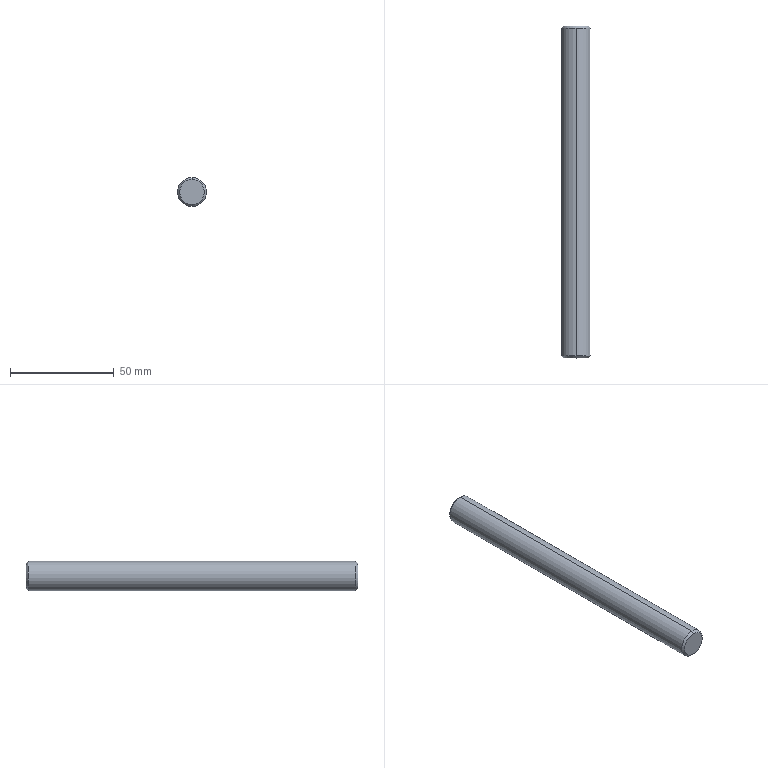Component | SolidWorks | AdjustingScrew9.26-3 | 1 solid | 8 faces | box 14 x 160 x 14 mm | volume 24588 mm3 | cone 4 | cylinder 2 | plane 2 | commonest cylinder face diameters 14 x2
build123d program:
from build123d import *

# Parameters (mm, degrees)
SKETCH1_R           = 7
BOSS_EXTRUDE1_DEPTH = 160
CHAMFER1_SIZE       = 1


with BuildPart() as part:
    # Sketch1 → Boss-Extrude1 (new body)
    with BuildSketch(Plane(origin=(0, 0, 0), x_dir=(1, 0, 0), z_dir=(0, 1, 0))):
        with Locations(Location((0, 0, 0), (0, 0, 270))):
            Circle(SKETCH1_R)
    extrude(amount=BOSS_EXTRUDE1_DEPTH)

    # Chamfer1
    chamfer1_edges = [part.edges().sort_by_distance(p)[0] for p in [
        (0, 0, -7),
        (0, 160, -7),
    ]]
    chamfer(chamfer1_edges, length=CHAMFER1_SIZE)


solid = part.part

# Placed as in the assembly
solid = solid.moved(Location((33.705, -428, 70.25), (0, 0, 0)))